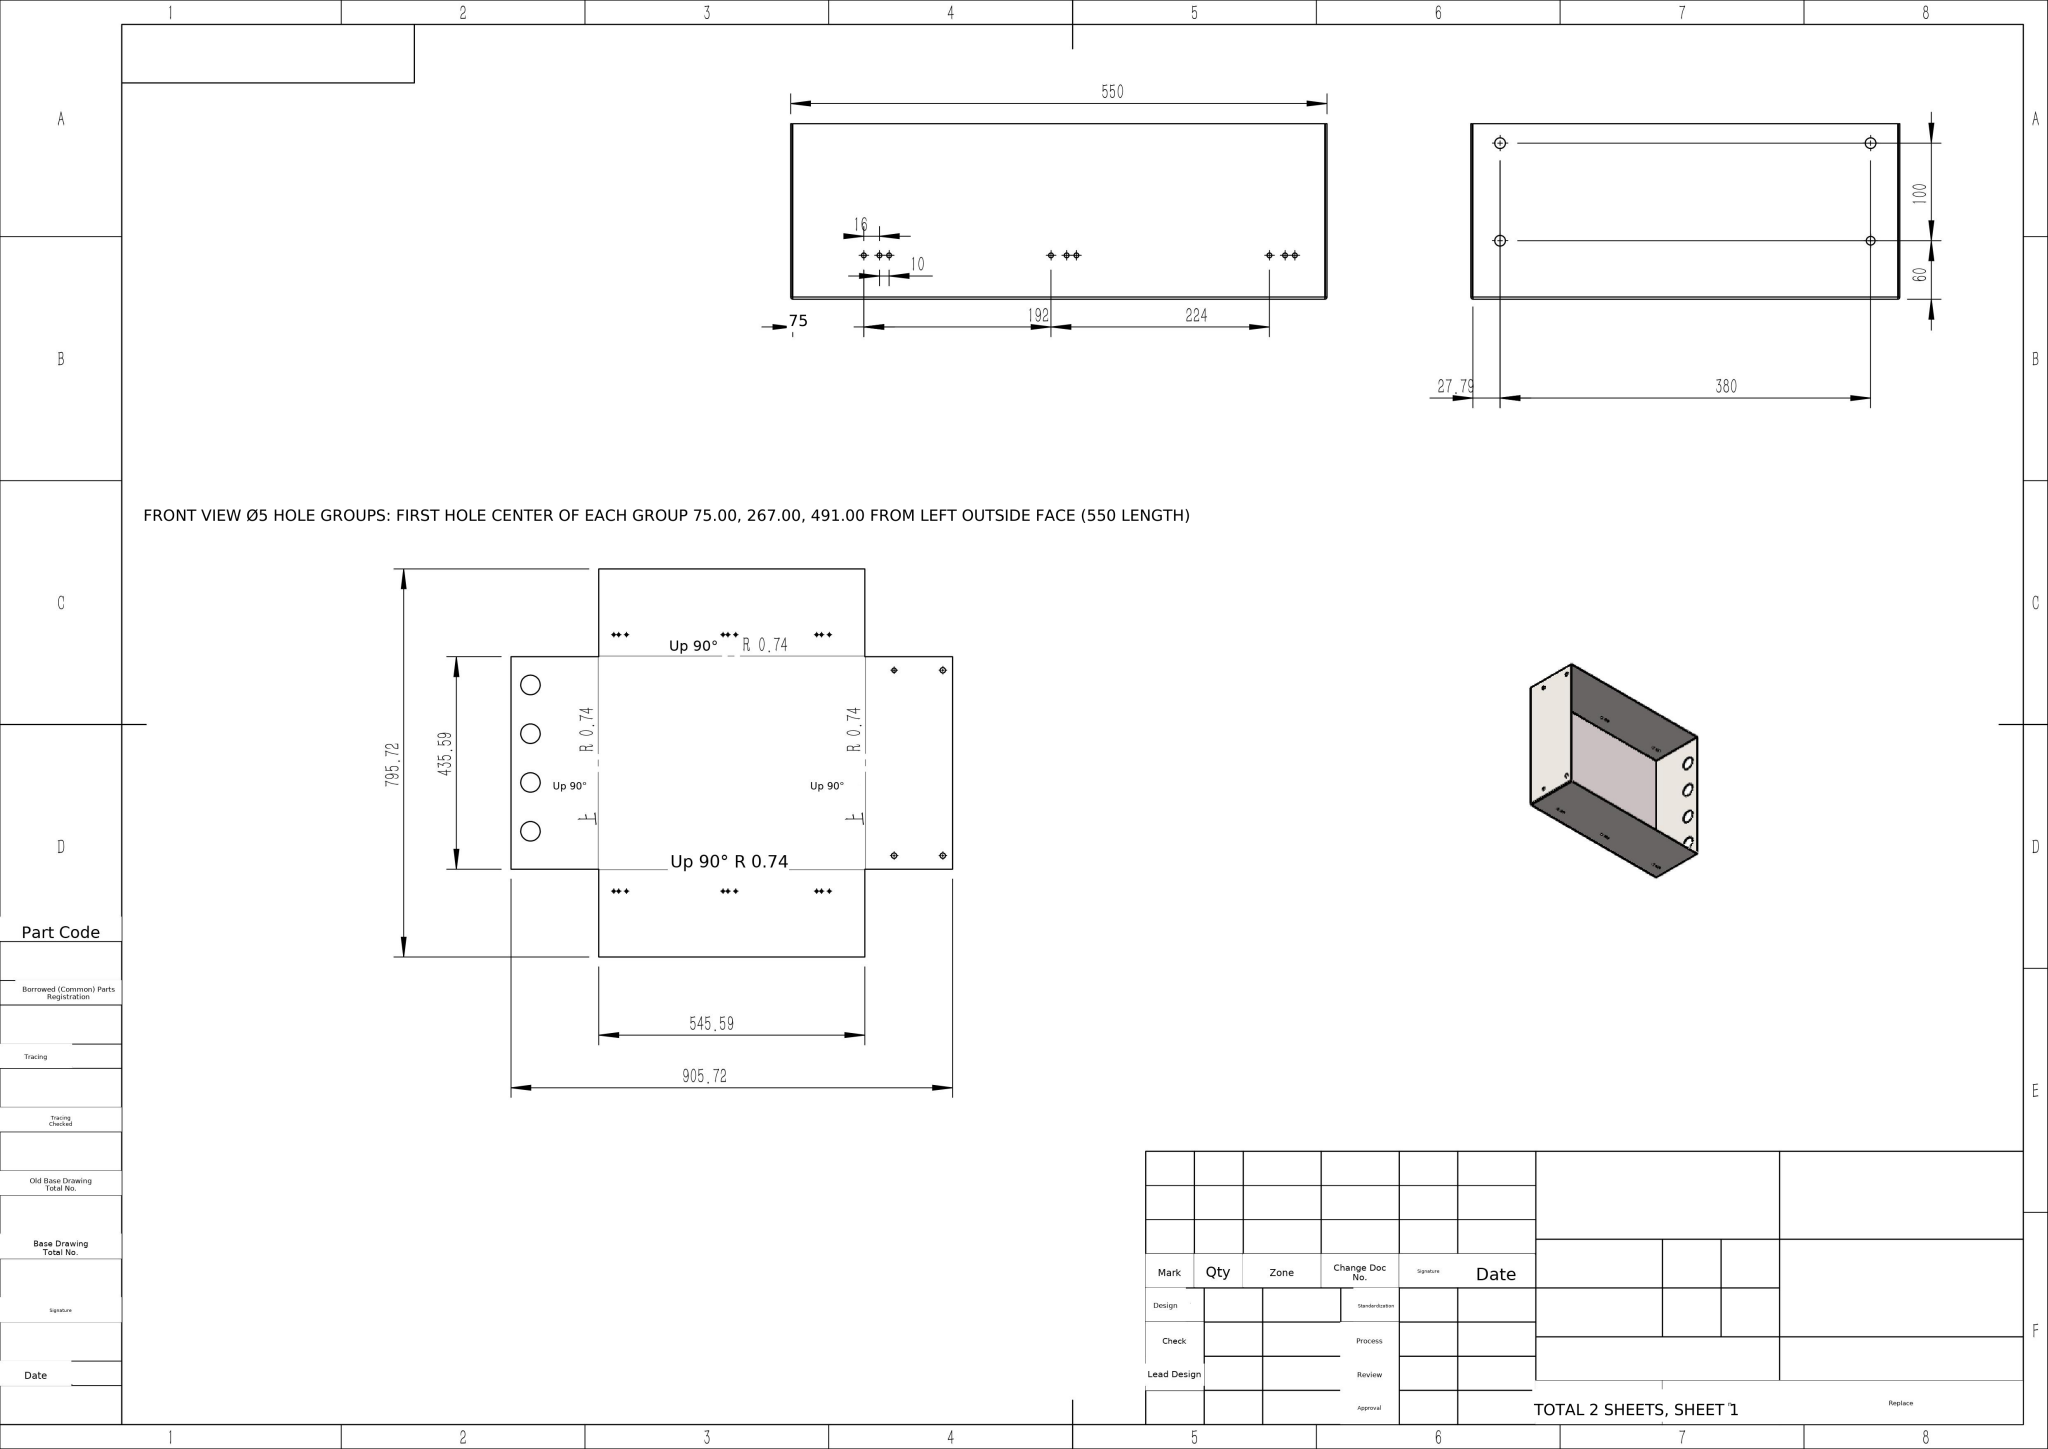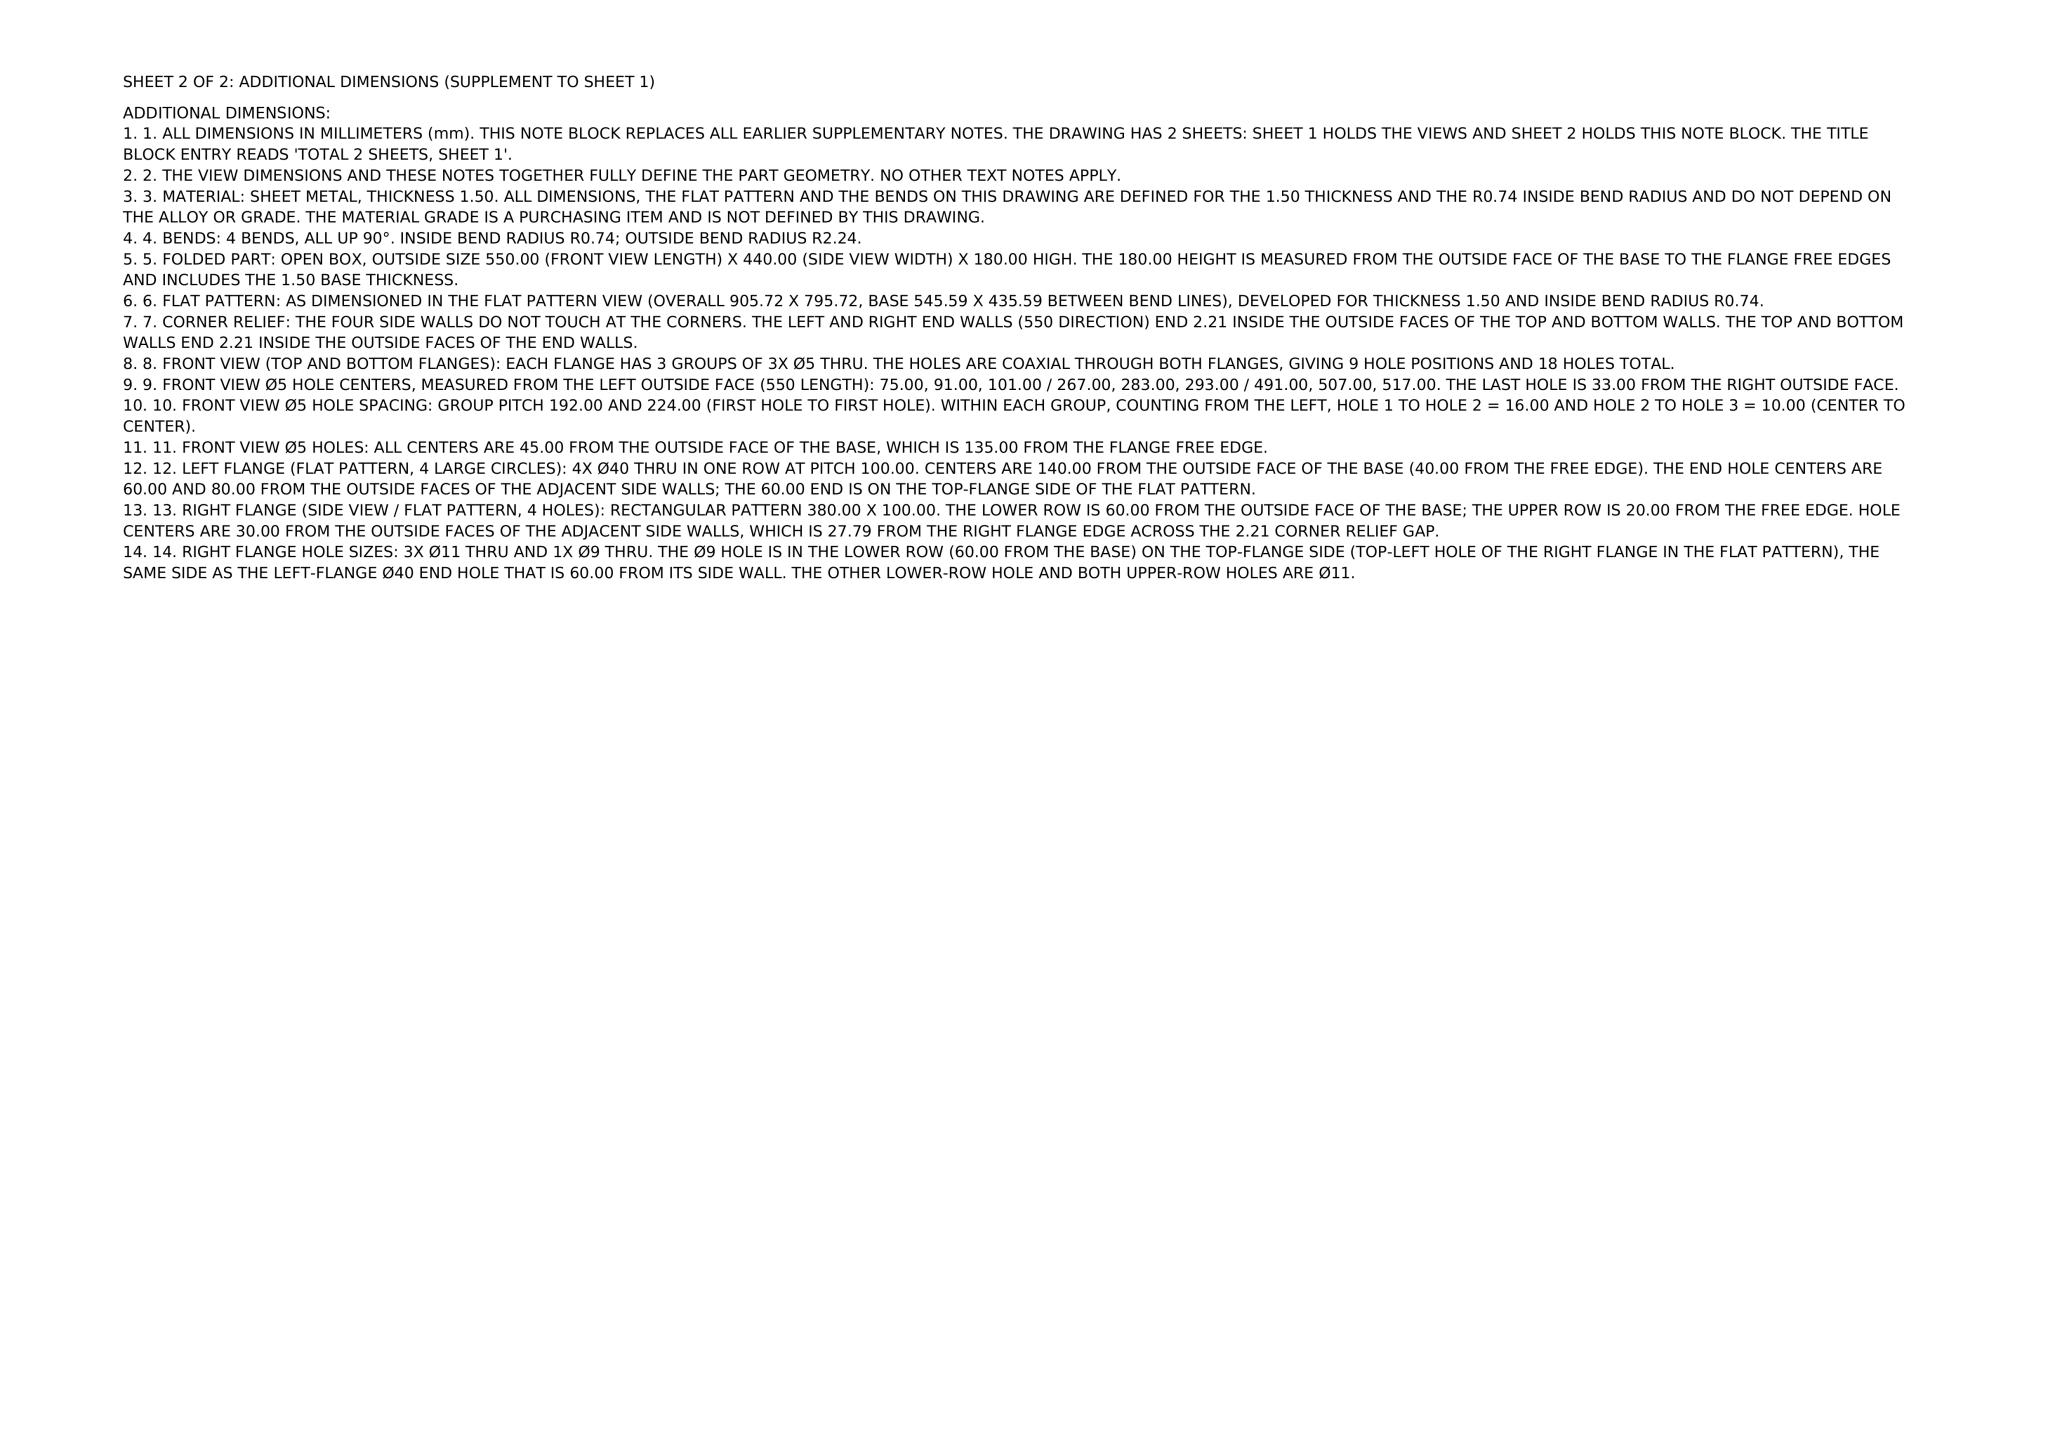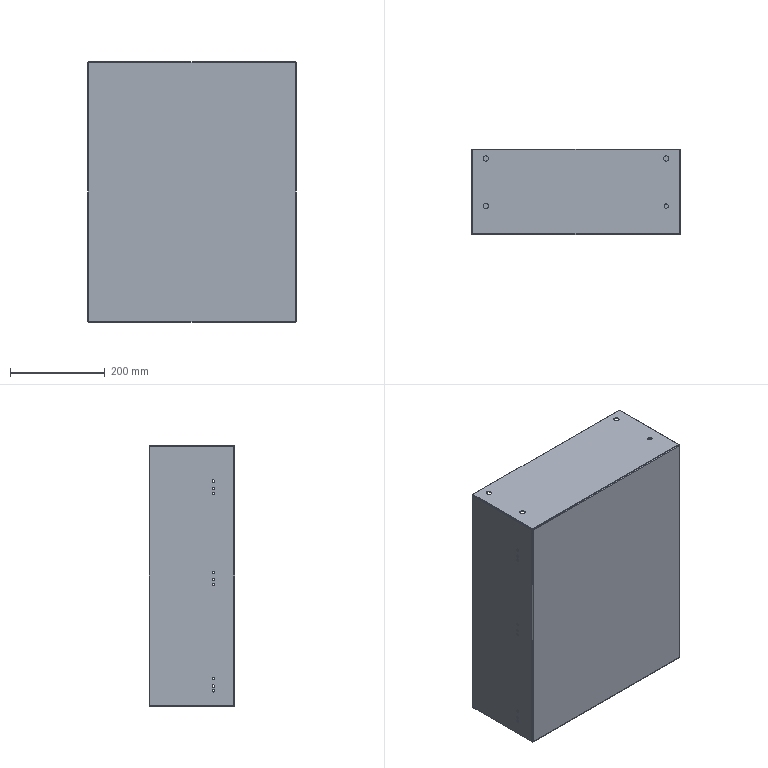Part | NX | mm | 1 solid | 90 faces | box 440 x 180 x 550 mm | volume 877917 mm3 | cylinder 60 | plane 22 | spline 8 | commonest cylinder face diameters 5 x36 40 x8 11 x6 4.473 x4 1.473 x4 9 x2